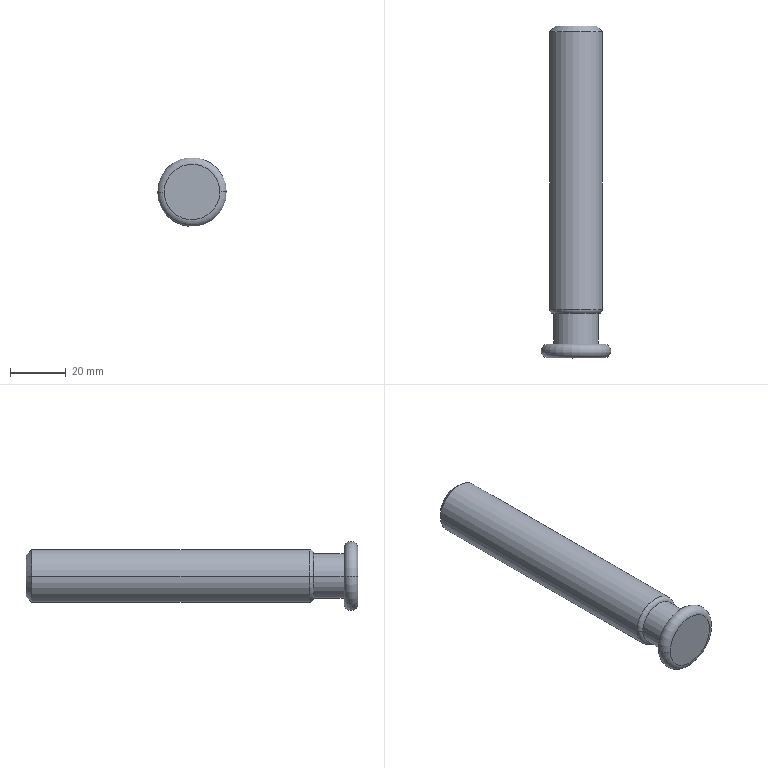Component | SolidWorks | 20mL - Glass Syringe-1_20mL - Glass Syringe Plunger-1 | 1 solid | 13 faces | box 25 x 119.5 x 25 mm | volume 33671 mm3 | cylinder 4 | torus 4 | plane 3 | cone 2 | commonest cylinder face diameters 19 x2 16 x2
build123d program:
from build123d import *


with BuildPart() as part:
    # Sketch1 → Revolve1 (revolve)
    with BuildSketch(Plane.XY, mode=Mode.PRIVATE) as revolve1_sk:
        with BuildLine():
            Line((0, 0), (0, 10))
            ThreePointArc((0, 10), (2.5, 12.5), (5, 10))
            Line((5, 10), (5, 8))
            Line((5, 8), (16, 8))
            ThreePointArc((16, 8), (16.439, 9.061), (17.5, 9.5))
            Line((17.5, 9.5), (117.5, 9.5))
            Line((117.5, 9.5), (119.5, 7.5))
            Line((119.5, 7.5), (119.5, 0))
            Line((119.5, 0), (0, 0))
        make_face()
    revolve(revolve1_sk.sketch.rotate(Axis((0, 0, 0), (1, 0, 0)), 90), axis=Axis((0, 0, 0), (1, 0, 0)))


solid = part.part

# Placed as in the assembly
solid = solid.moved(Location((417.806, 1211.5, -1928.012), (0, 0, 90)))
STEP:
#1=COLOUR_RGB('',0.7922,0.8196,0.9333);
#2=FILL_AREA_STYLE_COLOUR('',#1);
#3=FILL_AREA_STYLE('',(#2));
#4=SURFACE_STYLE_FILL_AREA(#3);
#5=SURFACE_SIDE_STYLE('',(#4));
#6=SURFACE_STYLE_USAGE(.BOTH.,#5);
#7=PRESENTATION_STYLE_ASSIGNMENT((#6));
#8=CARTESIAN_POINT('',(16.744,52.402,-75.903));
#9=VERTEX_POINT('',#8);
#10=CARTESIAN_POINT('',(16.154,52.402,-75.909));
#11=VERTEX_POINT('',#10);
#12=CARTESIAN_POINT('',(16.449,52.402,-75.906));
#13=DIRECTION('',(0.,-1.,0.));
#14=DIRECTION('',(1.,0.,0.009293));
#15=AXIS2_PLACEMENT_3D('',#12,#13,#14);
#16=CIRCLE('',#15,0.2953);
#17=EDGE_CURVE('',#9,#11,#16,.T.);
#18=ORIENTED_EDGE('',*,*,#17,.T.);
#19=CARTESIAN_POINT('',(16.075,52.323,-75.909));
#20=VERTEX_POINT('',#19);
#21=CARTESIAN_POINT('',(16.154,52.402,-75.909));
#22=DIRECTION('',(-0.7071,-0.7071,-0.006571));
#23=VECTOR('',#22,39.37);
#24=LINE('',#21,#23);
#25=EDGE_CURVE('',#11,#20,#24,.T.);
#26=ORIENTED_EDGE('',*,*,#25,.T.);
#27=CARTESIAN_POINT('',(16.823,52.323,-75.902));
#28=VERTEX_POINT('',#27);
#29=CARTESIAN_POINT('',(16.449,52.323,-75.906));
#30=DIRECTION('',(0.,-1.,0.));
#31=DIRECTION('',(1.,0.,0.009293));
#32=AXIS2_PLACEMENT_3D('',#29,#30,#31);
#33=CIRCLE('',#32,0.374);
#34=EDGE_CURVE('',#28,#20,#33,.T.);
#35=ORIENTED_EDGE('',*,*,#34,.F.);
#36=CARTESIAN_POINT('',(16.744,52.402,-75.903));
#37=DIRECTION('',(0.7071,-0.7071,0.006571));
#38=VECTOR('',#37,39.37);
#39=LINE('',#36,#38);
#40=EDGE_CURVE('',#9,#28,#39,.T.);
#41=ORIENTED_EDGE('',*,*,#40,.F.);
#42=EDGE_LOOP('',(#18,#26,#35,#41));
#43=FACE_OUTER_BOUND('',#42,.T.);
#44=CARTESIAN_POINT('',(16.449,52.402,-75.906));
#45=DIRECTION('',(0.,-1.,0.));
#46=DIRECTION('',(1.,0.,0.009293));
#47=AXIS2_PLACEMENT_3D('',#44,#45,#46);
#48=CONICAL_SURFACE('',#47,0.2953,0.7854);
#49=ADVANCED_FACE('',(#43),#48,.T.);
#50=ORIENTED_EDGE('',*,*,#34,.T.);
#51=CARTESIAN_POINT('',(16.075,48.386,-75.909));
#52=VERTEX_POINT('',#51);
#53=CARTESIAN_POINT('',(16.075,47.697,-75.909));
#54=DIRECTION('',(0.,-1.,0.));
#55=VECTOR('',#54,39.37);
#56=LINE('',#53,#55);
#57=EDGE_CURVE('',#20,#52,#56,.T.);
#58=ORIENTED_EDGE('',*,*,#57,.T.);
#59=CARTESIAN_POINT('',(16.823,48.386,-75.902));
#60=VERTEX_POINT('',#59);
#61=CARTESIAN_POINT('',(16.449,48.386,-75.906));
#62=DIRECTION('',(0.,-1.,0.));
#63=DIRECTION('',(1.,0.,0.009293));
#64=AXIS2_PLACEMENT_3D('',#61,#62,#63);
#65=CIRCLE('',#64,0.374);
#66=EDGE_CURVE('',#60,#52,#65,.T.);
#67=ORIENTED_EDGE('',*,*,#66,.F.);
#68=CARTESIAN_POINT('',(16.823,47.697,-75.902));
#69=DIRECTION('',(0.,-1.,0.));
#70=VECTOR('',#69,39.37);
#71=LINE('',#68,#70);
#72=EDGE_CURVE('',#28,#60,#71,.T.);
#73=ORIENTED_EDGE('',*,*,#72,.F.);
#74=EDGE_LOOP('',(#50,#58,#67,#73));
#75=FACE_OUTER_BOUND('',#74,.T.);
#76=CARTESIAN_POINT('',(16.449,47.697,-75.906));
#77=DIRECTION('',(0.,-1.,0.));
#78=DIRECTION('',(1.,0.,0.009293));
#79=AXIS2_PLACEMENT_3D('',#76,#77,#78);
#80=CYLINDRICAL_SURFACE('',#79,0.374);
#81=ADVANCED_FACE('',(#75),#80,.T.);
#82=ORIENTED_EDGE('',*,*,#66,.T.);
#83=CARTESIAN_POINT('',(16.134,48.327,-75.909));
#84=VERTEX_POINT('',#83);
#85=CARTESIAN_POINT('',(16.134,48.386,-75.909));
#86=DIRECTION('',(-0.009293,0.,1.));
#87=DIRECTION('',(1.,0.,0.009293));
#88=AXIS2_PLACEMENT_3D('',#85,#86,#87);
#89=CIRCLE('',#88,0.05906);
#90=EDGE_CURVE('',#52,#84,#89,.T.);
#91=ORIENTED_EDGE('',*,*,#90,.T.);
#92=CARTESIAN_POINT('',(16.764,48.327,-75.903));
#93=VERTEX_POINT('',#92);
#94=CARTESIAN_POINT('',(16.449,48.327,-75.906));
#95=DIRECTION('',(0.,-1.,0.));
#96=DIRECTION('',(1.,0.,0.009293));
#97=AXIS2_PLACEMENT_3D('',#94,#95,#96);
#98=CIRCLE('',#97,0.315);
#99=EDGE_CURVE('',#93,#84,#98,.T.);
#100=ORIENTED_EDGE('',*,*,#99,.F.);
#101=CARTESIAN_POINT('',(16.764,48.386,-75.903));
#102=DIRECTION('',(0.009293,-0.,-1.));
#103=DIRECTION('',(-1.,0.,-0.009293));
#104=AXIS2_PLACEMENT_3D('',#101,#102,#103);
#105=CIRCLE('',#104,0.05906);
#106=EDGE_CURVE('',#60,#93,#105,.T.);
#107=ORIENTED_EDGE('',*,*,#106,.F.);
#108=EDGE_LOOP('',(#82,#91,#100,#107));
#109=FACE_OUTER_BOUND('',#108,.T.);
#110=CARTESIAN_POINT('',(16.449,48.386,-75.906));
#111=DIRECTION('',(0.,-1.,0.));
#112=DIRECTION('',(1.,0.,0.009293));
#113=AXIS2_PLACEMENT_3D('',#110,#111,#112);
#114=TOROIDAL_SURFACE('',#113,0.315,0.05906);
#115=ADVANCED_FACE('',(#109),#114,.T.);
#116=ORIENTED_EDGE('',*,*,#99,.T.);
#117=CARTESIAN_POINT('',(16.134,47.894,-75.909));
#118=VERTEX_POINT('',#117);
#119=CARTESIAN_POINT('',(16.134,47.697,-75.909));
#120=DIRECTION('',(0.,-1.,0.));
#121=VECTOR('',#120,39.37);
#122=LINE('',#119,#121);
#123=EDGE_CURVE('',#84,#118,#122,.T.);
#124=ORIENTED_EDGE('',*,*,#123,.T.);
#125=CARTESIAN_POINT('',(16.764,47.894,-75.903));
#126=VERTEX_POINT('',#125);
#127=CARTESIAN_POINT('',(16.449,47.894,-75.906));
#128=DIRECTION('',(0.,-1.,0.));
#129=DIRECTION('',(1.,0.,0.009293));
#130=AXIS2_PLACEMENT_3D('',#127,#128,#129);
#131=CIRCLE('',#130,0.315);
#132=EDGE_CURVE('',#126,#118,#131,.T.);
#133=ORIENTED_EDGE('',*,*,#132,.F.);
#134=CARTESIAN_POINT('',(16.764,47.697,-75.903));
#135=DIRECTION('',(0.,-1.,0.));
#136=VECTOR('',#135,39.37);
#137=LINE('',#134,#136);
#138=EDGE_CURVE('',#93,#126,#137,.T.);
#139=ORIENTED_EDGE('',*,*,#138,.F.);
#140=EDGE_LOOP('',(#116,#124,#133,#139));
#141=FACE_OUTER_BOUND('',#140,.T.);
#142=CARTESIAN_POINT('',(16.449,47.697,-75.906));
#143=DIRECTION('',(0.,-1.,0.));
#144=DIRECTION('',(1.,0.,0.009293));
#145=AXIS2_PLACEMENT_3D('',#142,#143,#144);
#146=CYLINDRICAL_SURFACE('',#145,0.315);
#147=ADVANCED_FACE('',(#141),#146,.T.);
#148=CARTESIAN_POINT('',(16.843,47.894,-75.902));
#149=VERTEX_POINT('',#148);
#150=CARTESIAN_POINT('',(16.055,47.894,-75.91));
#151=VERTEX_POINT('',#150);
#152=CARTESIAN_POINT('',(16.449,47.894,-75.906));
#153=DIRECTION('',(0.,-1.,0.));
#154=DIRECTION('',(1.,0.,0.009293));
#155=AXIS2_PLACEMENT_3D('',#152,#153,#154);
#156=CIRCLE('',#155,0.3937);
#157=EDGE_CURVE('',#149,#151,#156,.T.);
#158=ORIENTED_EDGE('',*,*,#157,.T.);
#159=CARTESIAN_POINT('',(16.055,47.697,-75.91));
#160=VERTEX_POINT('',#159);
#161=CARTESIAN_POINT('',(16.055,47.795,-75.91));
#162=DIRECTION('',(-0.009293,0.,1.));
#163=DIRECTION('',(1.,0.,0.009293));
#164=AXIS2_PLACEMENT_3D('',#161,#162,#163);
#165=CIRCLE('',#164,0.09843);
#166=EDGE_CURVE('',#151,#160,#165,.T.);
#167=ORIENTED_EDGE('',*,*,#166,.T.);
#168=CARTESIAN_POINT('',(16.843,47.697,-75.902));
#169=VERTEX_POINT('',#168);
#170=CARTESIAN_POINT('',(16.449,47.697,-75.906));
#171=DIRECTION('',(0.,-1.,0.));
#172=DIRECTION('',(1.,0.,0.009293));
#173=AXIS2_PLACEMENT_3D('',#170,#171,#172);
#174=CIRCLE('',#173,0.3937);
#175=EDGE_CURVE('',#169,#160,#174,.T.);
#176=ORIENTED_EDGE('',*,*,#175,.F.);
#177=CARTESIAN_POINT('',(16.843,47.795,-75.902));
#178=DIRECTION('',(0.009293,-0.,-1.));
#179=DIRECTION('',(-1.,0.,-0.009293));
#180=AXIS2_PLACEMENT_3D('',#177,#178,#179);
#181=CIRCLE('',#180,0.09843);
#182=EDGE_CURVE('',#149,#169,#181,.T.);
#183=ORIENTED_EDGE('',*,*,#182,.F.);
#184=EDGE_LOOP('',(#158,#167,#176,#183));
#185=FACE_OUTER_BOUND('',#184,.T.);
#186=CARTESIAN_POINT('',(16.449,47.795,-75.906));
#187=DIRECTION('',(0.,-1.,0.));
#188=DIRECTION('',(1.,0.,0.009293));
#189=AXIS2_PLACEMENT_3D('',#186,#187,#188);
#190=TOROIDAL_SURFACE('',#189,0.3937,0.09843);
#191=ADVANCED_FACE('',(#185),#190,.T.);
#192=ORIENTED_EDGE('',*,*,#175,.T.);
#193=CARTESIAN_POINT('',(16.449,47.697,-75.906));
#194=DIRECTION('',(0.,-1.,0.));
#195=DIRECTION('',(1.,0.,0.009293));
#196=AXIS2_PLACEMENT_3D('',#193,#194,#195);
#197=CIRCLE('',#196,0.3937);
#198=EDGE_CURVE('',#160,#169,#197,.T.);
#199=ORIENTED_EDGE('',*,*,#198,.T.);
#200=EDGE_LOOP('',(#192,#199));
#201=FACE_OUTER_BOUND('',#200,.T.);
#202=CARTESIAN_POINT('',(16.449,47.697,-75.906));
#203=DIRECTION('',(-0.,1.,-0.));
#204=DIRECTION('',(-1.,-0.,-0.009293));
#205=AXIS2_PLACEMENT_3D('',#202,#203,#204);
#206=PLANE('',#205);
#207=ADVANCED_FACE('',(#201),#206,.F.);
#208=ORIENTED_EDGE('',*,*,#166,.F.);
#209=CARTESIAN_POINT('',(16.449,47.894,-75.906));
#210=DIRECTION('',(0.,-1.,0.));
#211=DIRECTION('',(1.,0.,0.009293));
#212=AXIS2_PLACEMENT_3D('',#209,#210,#211);
#213=CIRCLE('',#212,0.3937);
#214=EDGE_CURVE('',#151,#149,#213,.T.);
#215=ORIENTED_EDGE('',*,*,#214,.T.);
#216=ORIENTED_EDGE('',*,*,#182,.T.);
#217=ORIENTED_EDGE('',*,*,#198,.F.);
#218=EDGE_LOOP('',(#208,#215,#216,#217));
#219=FACE_OUTER_BOUND('',#218,.T.);
#220=CARTESIAN_POINT('',(16.449,47.795,-75.906));
#221=DIRECTION('',(0.,-1.,0.));
#222=DIRECTION('',(1.,0.,0.009293));
#223=AXIS2_PLACEMENT_3D('',#220,#221,#222);
#224=TOROIDAL_SURFACE('',#223,0.3937,0.09843);
#225=ADVANCED_FACE('',(#219),#224,.T.);
#226=ORIENTED_EDGE('',*,*,#157,.F.);
#227=ORIENTED_EDGE('',*,*,#214,.F.);
#228=EDGE_LOOP('',(#226,#227));
#229=FACE_OUTER_BOUND('',#228,.T.);
#230=ORIENTED_EDGE('',*,*,#132,.T.);
#231=CARTESIAN_POINT('',(16.449,47.894,-75.906));
#232=DIRECTION('',(0.,-1.,0.));
#233=DIRECTION('',(1.,0.,0.009293));
#234=AXIS2_PLACEMENT_3D('',#231,#232,#233);
#235=CIRCLE('',#234,0.315);
#236=EDGE_CURVE('',#118,#126,#235,.T.);
#237=ORIENTED_EDGE('',*,*,#236,.T.);
#238=EDGE_LOOP('',(#230,#237));
#239=FACE_BOUND('',#238,.T.);
#240=CARTESIAN_POINT('',(16.445,47.894,-75.512));
#241=DIRECTION('',(0.,-1.,0.));
#242=DIRECTION('',(1.,0.,0.009293));
#243=AXIS2_PLACEMENT_3D('',#240,#241,#242);
#244=PLANE('',#243);
#245=ADVANCED_FACE('',(#229,#239),#244,.F.);
#246=ORIENTED_EDGE('',*,*,#123,.F.);
#247=CARTESIAN_POINT('',(16.449,48.327,-75.906));
#248=DIRECTION('',(0.,-1.,0.));
#249=DIRECTION('',(1.,0.,0.009293));
#250=AXIS2_PLACEMENT_3D('',#247,#248,#249);
#251=CIRCLE('',#250,0.315);
#252=EDGE_CURVE('',#84,#93,#251,.T.);
#253=ORIENTED_EDGE('',*,*,#252,.T.);
#254=ORIENTED_EDGE('',*,*,#138,.T.);
#255=ORIENTED_EDGE('',*,*,#236,.F.);
#256=EDGE_LOOP('',(#246,#253,#254,#255));
#257=FACE_OUTER_BOUND('',#256,.T.);
#258=CARTESIAN_POINT('',(16.449,47.697,-75.906));
#259=DIRECTION('',(0.,-1.,0.));
#260=DIRECTION('',(1.,0.,0.009293));
#261=AXIS2_PLACEMENT_3D('',#258,#259,#260);
#262=CYLINDRICAL_SURFACE('',#261,0.315);
#263=ADVANCED_FACE('',(#257),#262,.T.);
#264=ORIENTED_EDGE('',*,*,#90,.F.);
#265=CARTESIAN_POINT('',(16.449,48.386,-75.906));
#266=DIRECTION('',(0.,-1.,0.));
#267=DIRECTION('',(1.,0.,0.009293));
#268=AXIS2_PLACEMENT_3D('',#265,#266,#267);
#269=CIRCLE('',#268,0.374);
#270=EDGE_CURVE('',#52,#60,#269,.T.);
#271=ORIENTED_EDGE('',*,*,#270,.T.);
#272=ORIENTED_EDGE('',*,*,#106,.T.);
#273=ORIENTED_EDGE('',*,*,#252,.F.);
#274=EDGE_LOOP('',(#264,#271,#272,#273));
#275=FACE_OUTER_BOUND('',#274,.T.);
#276=CARTESIAN_POINT('',(16.449,48.386,-75.906));
#277=DIRECTION('',(0.,-1.,0.));
#278=DIRECTION('',(1.,0.,0.009293));
#279=AXIS2_PLACEMENT_3D('',#276,#277,#278);
#280=TOROIDAL_SURFACE('',#279,0.315,0.05906);
#281=ADVANCED_FACE('',(#275),#280,.T.);
#282=ORIENTED_EDGE('',*,*,#57,.F.);
#283=CARTESIAN_POINT('',(16.449,52.323,-75.906));
#284=DIRECTION('',(0.,-1.,0.));
#285=DIRECTION('',(1.,0.,0.009293));
#286=AXIS2_PLACEMENT_3D('',#283,#284,#285);
#287=CIRCLE('',#286,0.374);
#288=EDGE_CURVE('',#20,#28,#287,.T.);
#289=ORIENTED_EDGE('',*,*,#288,.T.);
#290=ORIENTED_EDGE('',*,*,#72,.T.);
#291=ORIENTED_EDGE('',*,*,#270,.F.);
#292=EDGE_LOOP('',(#282,#289,#290,#291));
#293=FACE_OUTER_BOUND('',#292,.T.);
#294=CARTESIAN_POINT('',(16.449,47.697,-75.906));
#295=DIRECTION('',(0.,-1.,0.));
#296=DIRECTION('',(1.,0.,0.009293));
#297=AXIS2_PLACEMENT_3D('',#294,#295,#296);
#298=CYLINDRICAL_SURFACE('',#297,0.374);
#299=ADVANCED_FACE('',(#293),#298,.T.);
#300=ORIENTED_EDGE('',*,*,#25,.F.);
#301=CARTESIAN_POINT('',(16.449,52.402,-75.906));
#302=DIRECTION('',(0.,-1.,0.));
#303=DIRECTION('',(1.,0.,0.009293));
#304=AXIS2_PLACEMENT_3D('',#301,#302,#303);
#305=CIRCLE('',#304,0.2953);
#306=EDGE_CURVE('',#11,#9,#305,.T.);
#307=ORIENTED_EDGE('',*,*,#306,.T.);
#308=ORIENTED_EDGE('',*,*,#40,.T.);
#309=ORIENTED_EDGE('',*,*,#288,.F.);
#310=EDGE_LOOP('',(#300,#307,#308,#309));
#311=FACE_OUTER_BOUND('',#310,.T.);
#312=CARTESIAN_POINT('',(16.449,52.402,-75.906));
#313=DIRECTION('',(0.,-1.,0.));
#314=DIRECTION('',(1.,0.,0.009293));
#315=AXIS2_PLACEMENT_3D('',#312,#313,#314);
#316=CONICAL_SURFACE('',#315,0.2953,0.7854);
#317=ADVANCED_FACE('',(#311),#316,.T.);
#318=ORIENTED_EDGE('',*,*,#17,.F.);
#319=ORIENTED_EDGE('',*,*,#306,.F.);
#320=EDGE_LOOP('',(#318,#319));
#321=FACE_OUTER_BOUND('',#320,.T.);
#322=CARTESIAN_POINT('',(16.446,52.402,-75.611));
#323=DIRECTION('',(0.,-1.,0.));
#324=DIRECTION('',(1.,0.,0.009293));
#325=AXIS2_PLACEMENT_3D('',#322,#323,#324);
#326=PLANE('',#325);
#327=ADVANCED_FACE('',(#321),#326,.F.);
#328=CLOSED_SHELL('',(#49,#81,#115,#147,#191,#207,#225,#245,#263,#281,#299,#317,#327));
#329=MANIFOLD_SOLID_BREP('',#328);
#330=STYLED_ITEM('',(#7),#329);
#331=(LENGTH_UNIT()NAMED_UNIT(*)SI_UNIT($,.METRE.));
#332=LENGTH_MEASURE_WITH_UNIT(LENGTH_MEASURE(0.0254),#331);
#333=DIMENSIONAL_EXPONENTS(1.,0.,0.,0.,0.,0.,0.);
#334=(CONVERSION_BASED_UNIT('',#332)LENGTH_UNIT()NAMED_UNIT(#333));
#335=UNCERTAINTY_MEASURE_WITH_UNIT(LENGTH_MEASURE(0.00001),#334,'','');
#336=(NAMED_UNIT(*)PLANE_ANGLE_UNIT()SI_UNIT($,.RADIAN.));
#337=(NAMED_UNIT(*)SI_UNIT($,.STERADIAN.)SOLID_ANGLE_UNIT());
#338=(GEOMETRIC_REPRESENTATION_CONTEXT(3)GLOBAL_UNCERTAINTY_ASSIGNED_CONTEXT((#335))GLOBAL_UNIT_ASSIGNED_CONTEXT((#334,#336,#337))REPRESENTATION_CONTEXT('',''));
#339=MECHANICAL_DESIGN_GEOMETRIC_PRESENTATION_REPRESENTATION('',(#330),#338);
#340=CARTESIAN_POINT('',(0.,0.,0.));
#341=DIRECTION('',(0.,0.,1.));
#342=DIRECTION('',(1.,0.,0.));
#343=AXIS2_PLACEMENT_3D('',#340,#341,#342);
#344=(LENGTH_UNIT()NAMED_UNIT(*)SI_UNIT($,.METRE.));
#345=LENGTH_MEASURE_WITH_UNIT(LENGTH_MEASURE(0.0254),#344);
#346=DIMENSIONAL_EXPONENTS(1.,0.,0.,0.,0.,0.,0.);
#347=(CONVERSION_BASED_UNIT('',#345)LENGTH_UNIT()NAMED_UNIT(#346));
#348=UNCERTAINTY_MEASURE_WITH_UNIT(LENGTH_MEASURE(0.00001),#347,'','');
#349=(NAMED_UNIT(*)PLANE_ANGLE_UNIT()SI_UNIT($,.RADIAN.));
#350=(NAMED_UNIT(*)SI_UNIT($,.STERADIAN.)SOLID_ANGLE_UNIT());
#351=(GEOMETRIC_REPRESENTATION_CONTEXT(3)GLOBAL_UNCERTAINTY_ASSIGNED_CONTEXT((#348))GLOBAL_UNIT_ASSIGNED_CONTEXT((#347,#349,#350))REPRESENTATION_CONTEXT('',''));
#352=ADVANCED_BREP_SHAPE_REPRESENTATION('',(#329,#343),#351);
#353=PRESENTATION_LAYER_ASSIGNMENT('','',(#330));